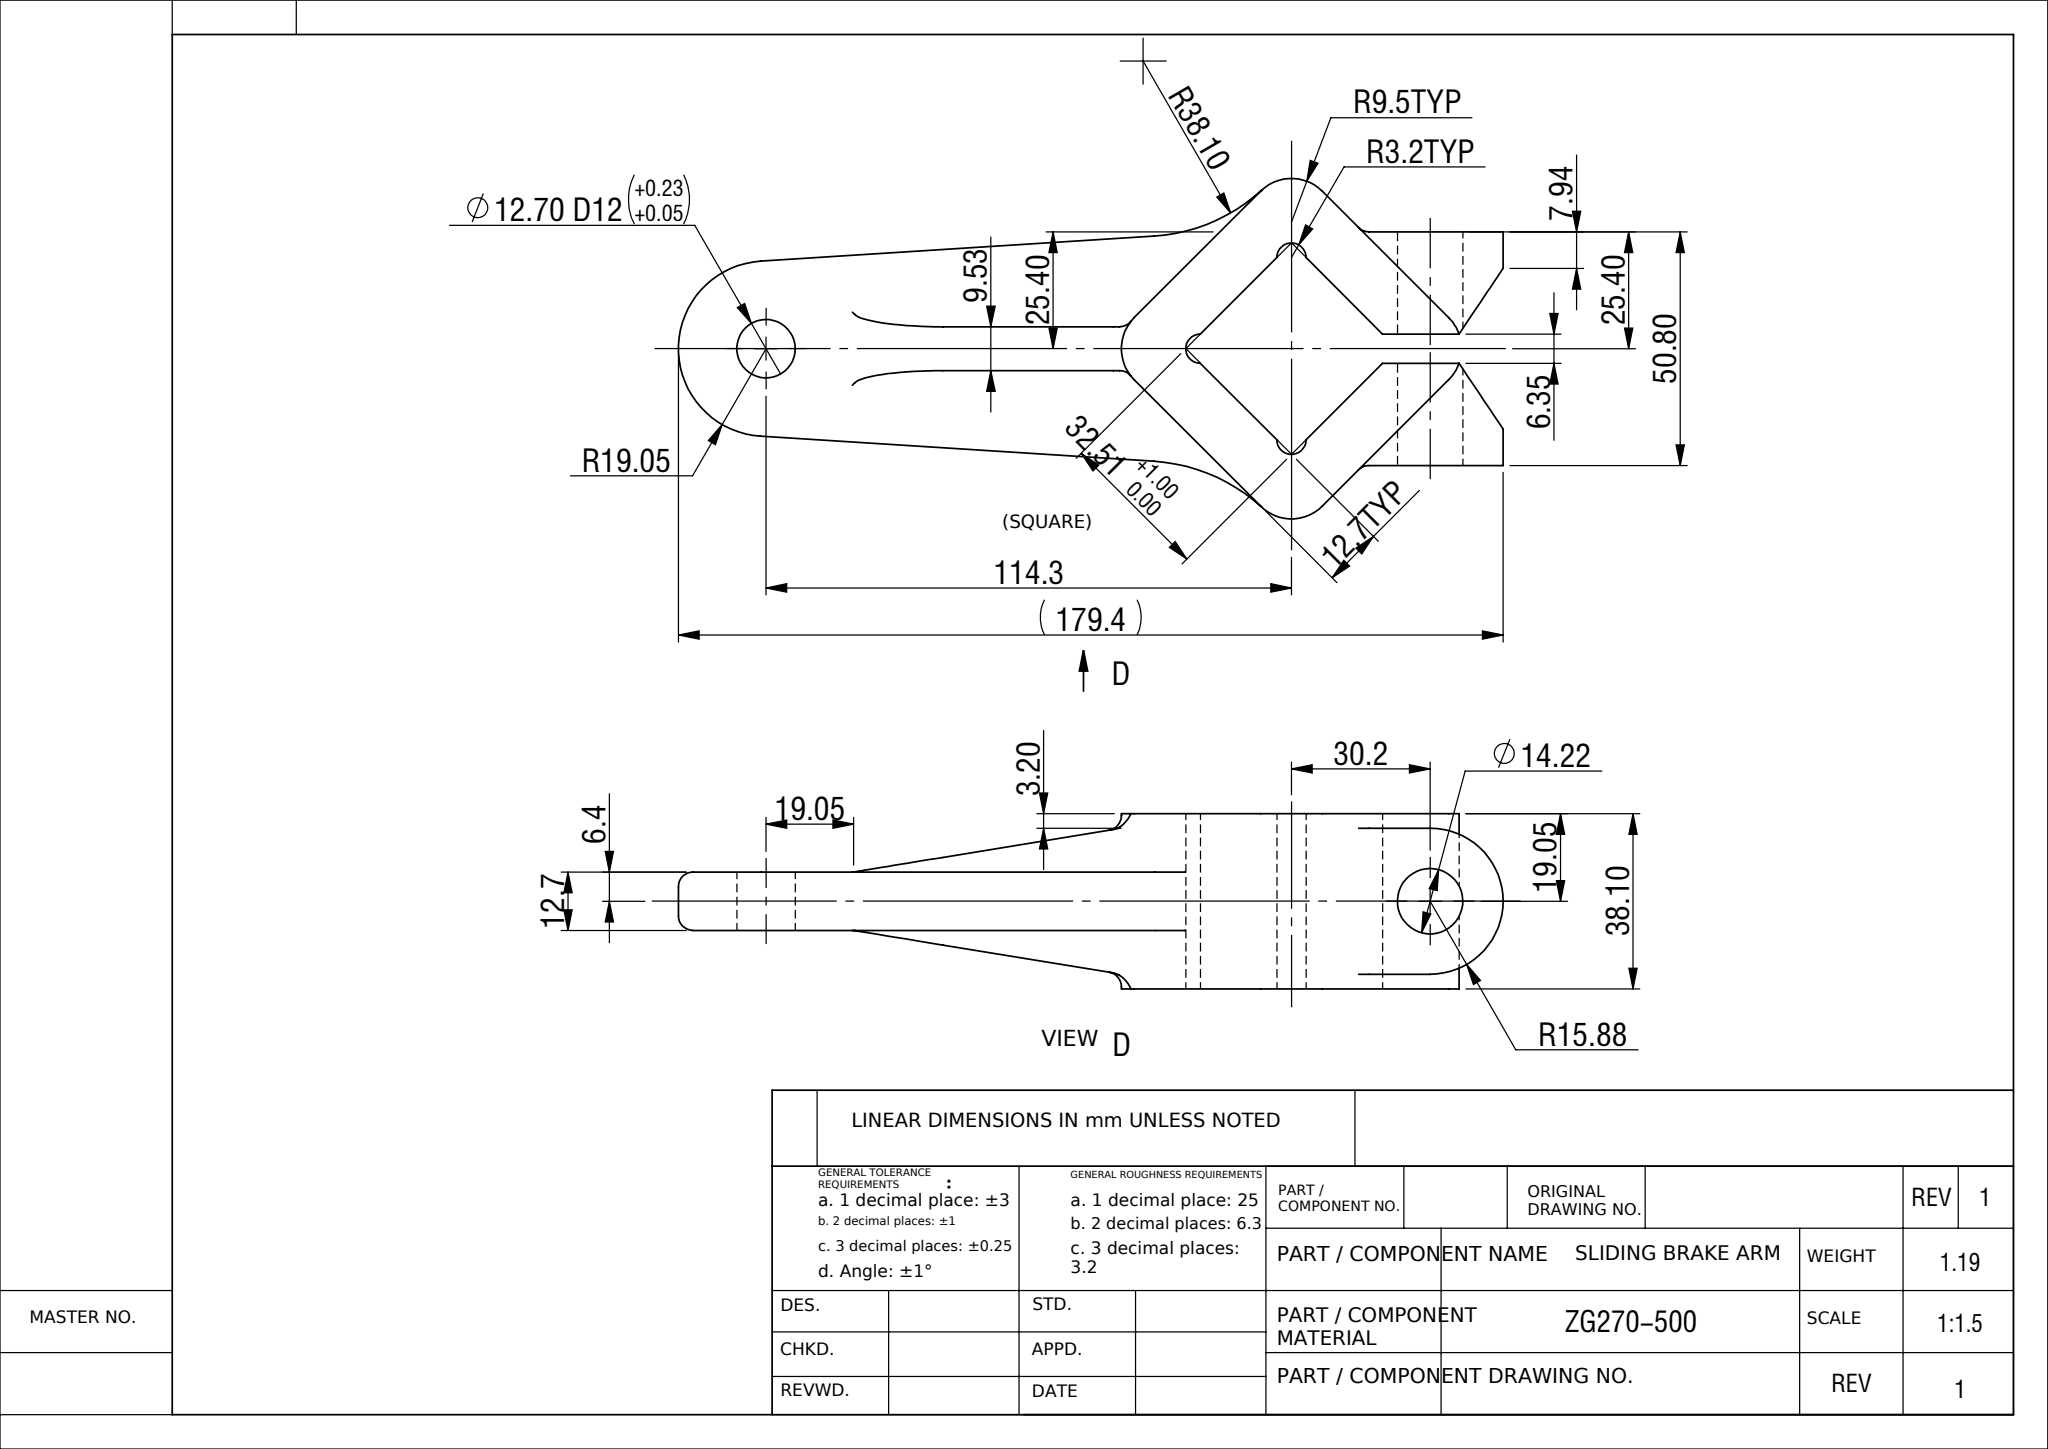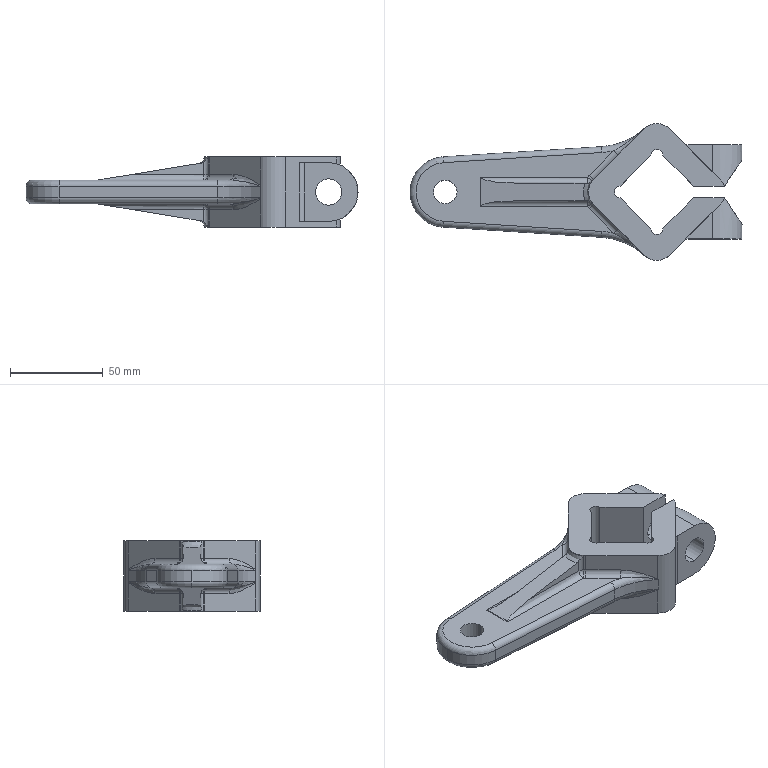Part | SolidWorks | drawing in inches | material ZG270-500 | 1 solid | 101 faces | box 179.39 x 74.01 x 38.1 mm | volume 152427 mm3 | cylinder 44 | plane 32 | torus 11 | spline 10 | sphere 4 | commonest cylinder face diameters 6.35 x23 19.05 x9 14.224 x4 12.7 x2 38.1 x2 31.75 x2 76.2 x2